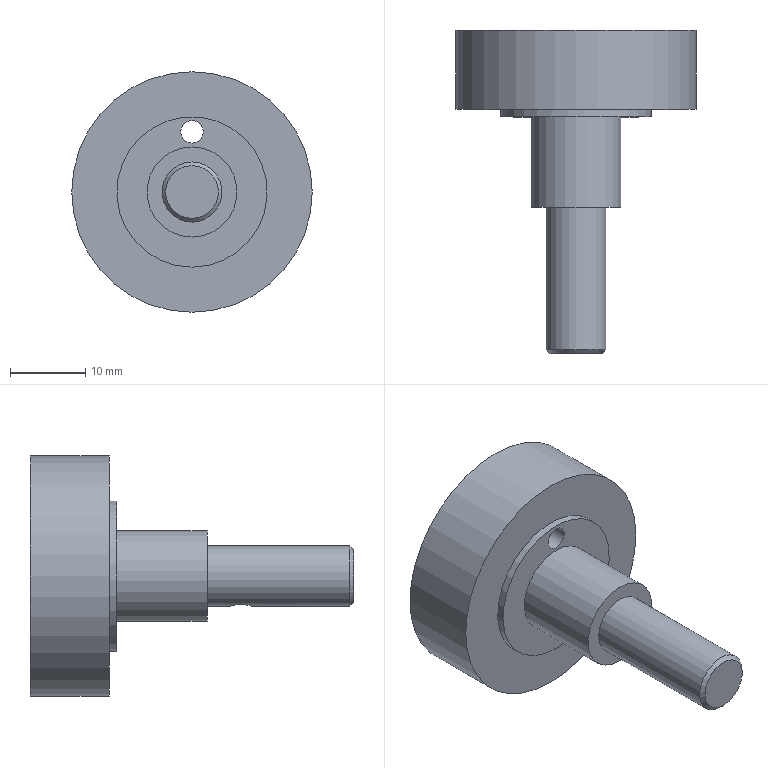Component | NX | ECCENTRIC_WHEEL | 1 solid | 14 faces | volume 10921 mm3 | cylinder 6 | plane 6 | cone 2 | commonest cylinder face diameters 12 x1 8 x1 32 x1 20 x1 3 x1 5 x1